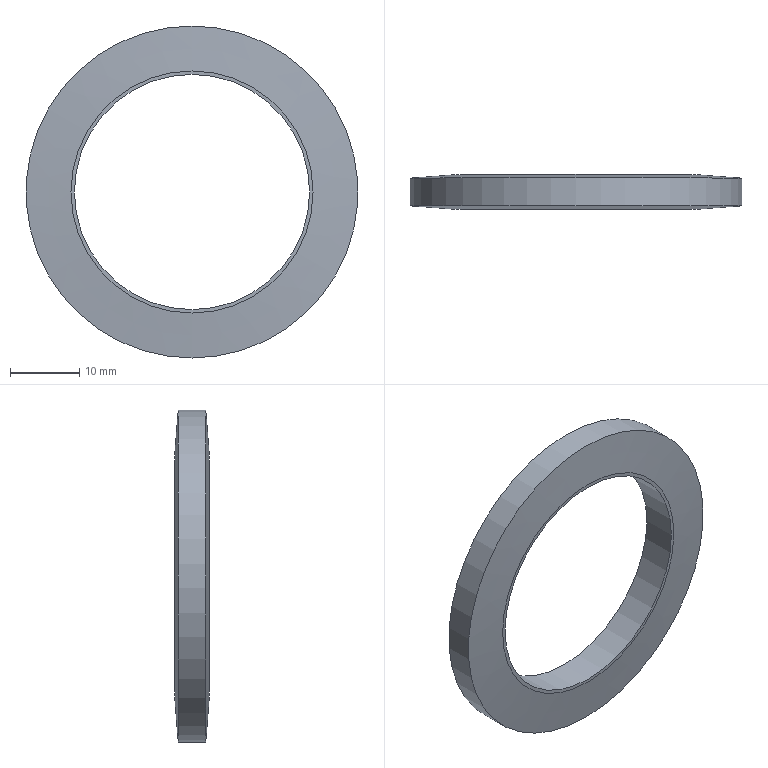Component | NX | FELT_RING_2 | 1 solid | 6 faces | box 48 x 5 x 48 mm | volume 4062 mm3 | cylinder 2 | plane 2 | cone 2 | commonest cylinder face diameters 48 x1 34 x1
STEP:
#1=CARTESIAN_POINT('',(0.,0.,0.));
#2=DIRECTION('',(0.,0.,1.));
#3=DIRECTION('',(1.,0.,0.));
#4=AXIS2_PLACEMENT_3D('',#1,#2,#3);
#5=CARTESIAN_POINT('',(378.803,-112.,-159.));
#6=VERTEX_POINT('',#5);
#7=CARTESIAN_POINT('',(378.803,-112.,-135.));
#8=DIRECTION('',(0.,-1.,0.));
#9=DIRECTION('',(0.,0.,-1.));
#10=AXIS2_PLACEMENT_3D('',#7,#8,#9);
#11=CIRCLE('',#10,24.);
#12=CARTESIAN_POINT('',(378.803,-116.5,-135.));
#13=DIRECTION('',(0.,1.,0.));
#14=DIRECTION('',(0.,0.,1.));
#15=AXIS2_PLACEMENT_3D('',#12,#13,#14);
#16=CYLINDRICAL_SURFACE('',#15,24.);
#17=CARTESIAN_POINT('',(9.425,4.5));
#18=DIRECTION('',(-1.,0.));
#19=VECTOR('',#18,1.);
#20=LINE('',#17,#19);
#21=(GEOMETRIC_REPRESENTATION_CONTEXT(2)PARAMETRIC_REPRESENTATION_CONTEXT()REPRESENTATION_CONTEXT('',''));
#22=DEFINITIONAL_REPRESENTATION('',(#20),#21);
#23=PCURVE('',#16,#22);
#24=CARTESIAN_POINT('',(378.803,-112.,-135.));
#25=DIRECTION('',(0.,-1.,0.));
#26=DIRECTION('',(0.,0.,-1.));
#27=AXIS2_PLACEMENT_3D('',#24,#25,#26);
#28=CONICAL_SURFACE('',#27,24.,1.494);
#29=CARTESIAN_POINT('',(0.,0.));
#30=DIRECTION('',(1.,0.));
#31=VECTOR('',#30,1.);
#32=LINE('',#29,#31);
#33=(GEOMETRIC_REPRESENTATION_CONTEXT(2)PARAMETRIC_REPRESENTATION_CONTEXT()REPRESENTATION_CONTEXT('',''));
#34=DEFINITIONAL_REPRESENTATION('',(#32),#33);
#35=PCURVE('',#28,#34);
#36=SURFACE_CURVE('',#11,(#23,#35),.PCURVE_S1.);
#37=EDGE_CURVE('',#6,#6,#36,.T.);
#38=ORIENTED_EDGE('',*,*,#37,.T.);
#39=CARTESIAN_POINT('',(378.803,-116.,-159.));
#40=VERTEX_POINT('',#39);
#41=CARTESIAN_POINT('',(378.803,-116.,-159.));
#42=CARTESIAN_POINT('',(378.803,-112.,-159.));
#43=B_SPLINE_CURVE_WITH_KNOTS('',1,(#41,#42),.UNSPECIFIED.,.F.,.F.,(2,2),(0.5,4.5),.PIECEWISE_BEZIER_KNOTS.);
#44=CARTESIAN_POINT('',(3.142,0.));
#45=DIRECTION('',(0.,1.));
#46=VECTOR('',#45,1.);
#47=LINE('',#44,#46);
#48=(GEOMETRIC_REPRESENTATION_CONTEXT(2)PARAMETRIC_REPRESENTATION_CONTEXT()REPRESENTATION_CONTEXT('',''));
#49=DEFINITIONAL_REPRESENTATION('',(#47),#48);
#50=PCURVE('',#16,#49);
#51=CARTESIAN_POINT('',(9.425,0.));
#52=DIRECTION('',(0.,1.));
#53=VECTOR('',#52,1.);
#54=LINE('',#51,#53);
#55=(GEOMETRIC_REPRESENTATION_CONTEXT(2)PARAMETRIC_REPRESENTATION_CONTEXT()REPRESENTATION_CONTEXT('',''));
#56=DEFINITIONAL_REPRESENTATION('',(#54),#55);
#57=PCURVE('',#16,#56);
#58=SEAM_CURVE('',#43,(#50,#57),.PCURVE_S1.);
#59=EDGE_CURVE('',#40,#6,#58,.T.);
#60=ORIENTED_EDGE('',*,*,#59,.F.);
#61=CARTESIAN_POINT('',(378.803,-116.,-135.));
#62=DIRECTION('',(0.,1.,0.));
#63=DIRECTION('',(0.,0.,-1.));
#64=AXIS2_PLACEMENT_3D('',#61,#62,#63);
#65=CIRCLE('',#64,24.);
#66=CARTESIAN_POINT('',(3.142,0.5));
#67=DIRECTION('',(1.,0.));
#68=VECTOR('',#67,1.);
#69=LINE('',#66,#68);
#70=(GEOMETRIC_REPRESENTATION_CONTEXT(2)PARAMETRIC_REPRESENTATION_CONTEXT()REPRESENTATION_CONTEXT('',''));
#71=DEFINITIONAL_REPRESENTATION('',(#69),#70);
#72=PCURVE('',#16,#71);
#73=CARTESIAN_POINT('',(378.803,-116.5,-135.));
#74=DIRECTION('',(0.,1.,0.));
#75=DIRECTION('',(0.,0.,1.));
#76=AXIS2_PLACEMENT_3D('',#73,#74,#75);
#77=CONICAL_SURFACE('',#76,17.5,1.494);
#78=CARTESIAN_POINT('',(3.142,0.5));
#79=DIRECTION('',(1.,0.));
#80=VECTOR('',#79,1.);
#81=LINE('',#78,#80);
#82=(GEOMETRIC_REPRESENTATION_CONTEXT(2)PARAMETRIC_REPRESENTATION_CONTEXT()REPRESENTATION_CONTEXT('',''));
#83=DEFINITIONAL_REPRESENTATION('',(#81),#82);
#84=PCURVE('',#77,#83);
#85=SURFACE_CURVE('',#65,(#72,#84),.PCURVE_S1.);
#86=EDGE_CURVE('',#40,#40,#85,.T.);
#87=ORIENTED_EDGE('',*,*,#86,.T.);
#88=ORIENTED_EDGE('',*,*,#59,.T.);
#89=EDGE_LOOP('',(#38,#60,#87,#88));
#90=FACE_BOUND('',#89,.T.);
#91=ADVANCED_FACE('',(#90),#16,.T.);
#92=CARTESIAN_POINT('',(395.803,-116.5,-135.));
#93=VERTEX_POINT('',#92);
#94=CARTESIAN_POINT('',(378.803,-116.5,-135.));
#95=DIRECTION('',(0.,-1.,0.));
#96=DIRECTION('',(1.,0.,0.));
#97=AXIS2_PLACEMENT_3D('',#94,#95,#96);
#98=CIRCLE('',#97,17.);
#99=CARTESIAN_POINT('',(378.803,-116.5,-135.));
#100=DIRECTION('',(0.,1.,0.));
#101=DIRECTION('',(0.,0.,1.));
#102=AXIS2_PLACEMENT_3D('',#99,#100,#101);
#103=CYLINDRICAL_SURFACE('',#102,17.);
#104=CARTESIAN_POINT('',(7.854,0.));
#105=DIRECTION('',(-1.,0.));
#106=VECTOR('',#105,1.);
#107=LINE('',#104,#106);
#108=(GEOMETRIC_REPRESENTATION_CONTEXT(2)PARAMETRIC_REPRESENTATION_CONTEXT()REPRESENTATION_CONTEXT('',''));
#109=DEFINITIONAL_REPRESENTATION('',(#107),#108);
#110=PCURVE('',#103,#109);
#111=CARTESIAN_POINT('',(378.803,-116.5,-135.));
#112=DIRECTION('',(0.,-1.,0.));
#113=DIRECTION('',(0.,0.,-1.));
#114=AXIS2_PLACEMENT_3D('',#111,#112,#113);
#115=PLANE('',#114);
#116=CARTESIAN_POINT('',(0.,0.));
#117=DIRECTION('',(0.,1.));
#118=AXIS2_PLACEMENT_2D('',#116,#117);
#119=CIRCLE('',#118,17.);
#120=(GEOMETRIC_REPRESENTATION_CONTEXT(2)PARAMETRIC_REPRESENTATION_CONTEXT()REPRESENTATION_CONTEXT('',''));
#121=DEFINITIONAL_REPRESENTATION('',(#119),#120);
#122=PCURVE('',#115,#121);
#123=SURFACE_CURVE('',#98,(#110,#122),.PCURVE_S1.);
#124=EDGE_CURVE('',#93,#93,#123,.T.);
#125=ORIENTED_EDGE('',*,*,#124,.F.);
#126=CARTESIAN_POINT('',(395.803,-111.5,-135.));
#127=VERTEX_POINT('',#126);
#128=CARTESIAN_POINT('',(395.803,-116.5,-135.));
#129=CARTESIAN_POINT('',(395.803,-111.5,-135.));
#130=B_SPLINE_CURVE_WITH_KNOTS('',1,(#128,#129),.UNSPECIFIED.,.F.,.F.,(2,2),(0.,5.),.PIECEWISE_BEZIER_KNOTS.);
#131=CARTESIAN_POINT('',(7.854,0.));
#132=DIRECTION('',(0.,1.));
#133=VECTOR('',#132,1.);
#134=LINE('',#131,#133);
#135=(GEOMETRIC_REPRESENTATION_CONTEXT(2)PARAMETRIC_REPRESENTATION_CONTEXT()REPRESENTATION_CONTEXT('',''));
#136=DEFINITIONAL_REPRESENTATION('',(#134),#135);
#137=PCURVE('',#103,#136);
#138=CARTESIAN_POINT('',(1.571,0.));
#139=DIRECTION('',(0.,1.));
#140=VECTOR('',#139,1.);
#141=LINE('',#138,#140);
#142=(GEOMETRIC_REPRESENTATION_CONTEXT(2)PARAMETRIC_REPRESENTATION_CONTEXT()REPRESENTATION_CONTEXT('',''));
#143=DEFINITIONAL_REPRESENTATION('',(#141),#142);
#144=PCURVE('',#103,#143);
#145=SEAM_CURVE('',#130,(#137,#144),.PCURVE_S1.);
#146=EDGE_CURVE('',#93,#127,#145,.T.);
#147=ORIENTED_EDGE('',*,*,#146,.T.);
#148=CARTESIAN_POINT('',(378.803,-111.5,-135.));
#149=DIRECTION('',(0.,-1.,0.));
#150=DIRECTION('',(1.,0.,0.));
#151=AXIS2_PLACEMENT_3D('',#148,#149,#150);
#152=CIRCLE('',#151,17.);
#153=CARTESIAN_POINT('',(7.854,5.));
#154=DIRECTION('',(-1.,0.));
#155=VECTOR('',#154,1.);
#156=LINE('',#153,#155);
#157=(GEOMETRIC_REPRESENTATION_CONTEXT(2)PARAMETRIC_REPRESENTATION_CONTEXT()REPRESENTATION_CONTEXT('',''));
#158=DEFINITIONAL_REPRESENTATION('',(#156),#157);
#159=PCURVE('',#103,#158);
#160=CARTESIAN_POINT('',(378.803,-111.5,-135.));
#161=DIRECTION('',(0.,-1.,0.));
#162=DIRECTION('',(0.,0.,-1.));
#163=AXIS2_PLACEMENT_3D('',#160,#161,#162);
#164=PLANE('',#163);
#165=CARTESIAN_POINT('',(0.,0.));
#166=DIRECTION('',(0.,1.));
#167=AXIS2_PLACEMENT_2D('',#165,#166);
#168=CIRCLE('',#167,17.);
#169=(GEOMETRIC_REPRESENTATION_CONTEXT(2)PARAMETRIC_REPRESENTATION_CONTEXT()REPRESENTATION_CONTEXT('',''));
#170=DEFINITIONAL_REPRESENTATION('',(#168),#169);
#171=PCURVE('',#164,#170);
#172=SURFACE_CURVE('',#152,(#159,#171),.PCURVE_S1.);
#173=EDGE_CURVE('',#127,#127,#172,.T.);
#174=ORIENTED_EDGE('',*,*,#173,.T.);
#175=ORIENTED_EDGE('',*,*,#146,.F.);
#176=EDGE_LOOP('',(#125,#147,#174,#175));
#177=FACE_BOUND('',#176,.F.);
#178=ADVANCED_FACE('',(#177),#103,.F.);
#179=CARTESIAN_POINT('',(378.803,-116.5,-152.5));
#180=VERTEX_POINT('',#179);
#181=CARTESIAN_POINT('',(378.803,-116.5,-135.));
#182=DIRECTION('',(0.,-1.,0.));
#183=DIRECTION('',(0.,0.,-1.));
#184=AXIS2_PLACEMENT_3D('',#181,#182,#183);
#185=CIRCLE('',#184,17.5);
#186=CARTESIAN_POINT('',(0.,0.));
#187=DIRECTION('',(1.,0.));
#188=AXIS2_PLACEMENT_2D('',#186,#187);
#189=CIRCLE('',#188,17.5);
#190=(GEOMETRIC_REPRESENTATION_CONTEXT(2)PARAMETRIC_REPRESENTATION_CONTEXT()REPRESENTATION_CONTEXT('',''));
#191=DEFINITIONAL_REPRESENTATION('',(#189),#190);
#192=PCURVE('',#115,#191);
#193=CARTESIAN_POINT('',(9.425,0.));
#194=DIRECTION('',(-1.,0.));
#195=VECTOR('',#194,1.);
#196=LINE('',#193,#195);
#197=(GEOMETRIC_REPRESENTATION_CONTEXT(2)PARAMETRIC_REPRESENTATION_CONTEXT()REPRESENTATION_CONTEXT('',''));
#198=DEFINITIONAL_REPRESENTATION('',(#196),#197);
#199=PCURVE('',#77,#198);
#200=SURFACE_CURVE('',#185,(#192,#199),.PCURVE_S1.);
#201=EDGE_CURVE('',#180,#180,#200,.T.);
#202=ORIENTED_EDGE('',*,*,#201,.T.);
#203=EDGE_LOOP('',(#202));
#204=FACE_BOUND('',#203,.T.);
#205=ORIENTED_EDGE('',*,*,#124,.F.);
#206=EDGE_LOOP('',(#205));
#207=FACE_BOUND('',#206,.T.);
#208=ADVANCED_FACE('',(#204,#207),#115,.T.);
#209=CARTESIAN_POINT('',(378.803,-111.5,-152.5));
#210=VERTEX_POINT('',#209);
#211=CARTESIAN_POINT('',(378.803,-111.5,-135.));
#212=DIRECTION('',(0.,1.,0.));
#213=DIRECTION('',(0.,0.,-1.));
#214=AXIS2_PLACEMENT_3D('',#211,#212,#213);
#215=CIRCLE('',#214,17.5);
#216=CARTESIAN_POINT('',(17.5,0.));
#217=CARTESIAN_POINT('',(17.5,-30.311));
#218=CARTESIAN_POINT('',(-8.75,-15.155));
#219=CARTESIAN_POINT('',(-35.,-0.));
#220=CARTESIAN_POINT('',(-8.75,15.155));
#221=CARTESIAN_POINT('',(17.5,30.311));
#222=CARTESIAN_POINT('',(17.5,0.));
#223=(BOUNDED_CURVE()B_SPLINE_CURVE(2,(#216,#217,#218,#219,#220,#221,#222),.UNSPECIFIED.,.T.,.F.)B_SPLINE_CURVE_WITH_KNOTS((1,2,2,2,2,1),(-2.094,0.,2.094,4.189,6.283,8.378),.UNSPECIFIED.)CURVE()GEOMETRIC_REPRESENTATION_ITEM()RATIONAL_B_SPLINE_CURVE((1.,0.5,1.,0.5,1.,0.5,1.))REPRESENTATION_ITEM(''));
#224=(GEOMETRIC_REPRESENTATION_CONTEXT(2)PARAMETRIC_REPRESENTATION_CONTEXT()REPRESENTATION_CONTEXT('',''));
#225=DEFINITIONAL_REPRESENTATION('',(#223),#224);
#226=PCURVE('',#164,#225);
#227=CARTESIAN_POINT('',(6.283,-0.5));
#228=DIRECTION('',(-1.,0.));
#229=VECTOR('',#228,1.);
#230=LINE('',#227,#229);
#231=(GEOMETRIC_REPRESENTATION_CONTEXT(2)PARAMETRIC_REPRESENTATION_CONTEXT()REPRESENTATION_CONTEXT('',''));
#232=DEFINITIONAL_REPRESENTATION('',(#230),#231);
#233=PCURVE('',#28,#232);
#234=SURFACE_CURVE('',#215,(#226,#233),.PCURVE_S1.);
#235=EDGE_CURVE('',#210,#210,#234,.T.);
#236=ORIENTED_EDGE('',*,*,#235,.T.);
#237=EDGE_LOOP('',(#236));
#238=FACE_BOUND('',#237,.T.);
#239=ORIENTED_EDGE('',*,*,#173,.T.);
#240=EDGE_LOOP('',(#239));
#241=FACE_BOUND('',#240,.T.);
#242=ADVANCED_FACE('',(#238,#241),#164,.F.);
#243=ORIENTED_EDGE('',*,*,#86,.F.);
#244=CARTESIAN_POINT('',(378.803,-116.5,-152.5));
#245=CARTESIAN_POINT('',(378.803,-116.,-159.));
#246=B_SPLINE_CURVE_WITH_KNOTS('',1,(#244,#245),.UNSPECIFIED.,.F.,.F.,(2,2),(0.,6.519),.PIECEWISE_BEZIER_KNOTS.);
#247=CARTESIAN_POINT('',(3.142,0.));
#248=DIRECTION('',(0.,1.));
#249=VECTOR('',#248,1.);
#250=LINE('',#247,#249);
#251=(GEOMETRIC_REPRESENTATION_CONTEXT(2)PARAMETRIC_REPRESENTATION_CONTEXT()REPRESENTATION_CONTEXT('',''));
#252=DEFINITIONAL_REPRESENTATION('',(#250),#251);
#253=PCURVE('',#77,#252);
#254=CARTESIAN_POINT('',(9.425,0.));
#255=DIRECTION('',(0.,1.));
#256=VECTOR('',#255,1.);
#257=LINE('',#254,#256);
#258=(GEOMETRIC_REPRESENTATION_CONTEXT(2)PARAMETRIC_REPRESENTATION_CONTEXT()REPRESENTATION_CONTEXT('',''));
#259=DEFINITIONAL_REPRESENTATION('',(#257),#258);
#260=PCURVE('',#77,#259);
#261=SEAM_CURVE('',#246,(#253,#260),.PCURVE_S1.);
#262=EDGE_CURVE('',#180,#40,#261,.T.);
#263=ORIENTED_EDGE('',*,*,#262,.F.);
#264=ORIENTED_EDGE('',*,*,#201,.F.);
#265=ORIENTED_EDGE('',*,*,#262,.T.);
#266=EDGE_LOOP('',(#243,#263,#264,#265));
#267=FACE_BOUND('',#266,.T.);
#268=ADVANCED_FACE('',(#267),#77,.T.);
#269=ORIENTED_EDGE('',*,*,#235,.F.);
#270=CARTESIAN_POINT('',(378.803,-111.5,-152.5));
#271=CARTESIAN_POINT('',(378.803,-112.,-159.));
#272=B_SPLINE_CURVE_WITH_KNOTS('',1,(#270,#271),.UNSPECIFIED.,.F.,.F.,(2,2),(-6.519,0.),.PIECEWISE_BEZIER_KNOTS.);
#273=CARTESIAN_POINT('',(6.283,0.));
#274=DIRECTION('',(0.,1.));
#275=VECTOR('',#274,1.);
#276=LINE('',#273,#275);
#277=(GEOMETRIC_REPRESENTATION_CONTEXT(2)PARAMETRIC_REPRESENTATION_CONTEXT()REPRESENTATION_CONTEXT('',''));
#278=DEFINITIONAL_REPRESENTATION('',(#276),#277);
#279=PCURVE('',#28,#278);
#280=CARTESIAN_POINT('',(0.,0.));
#281=DIRECTION('',(0.,1.));
#282=VECTOR('',#281,1.);
#283=LINE('',#280,#282);
#284=(GEOMETRIC_REPRESENTATION_CONTEXT(2)PARAMETRIC_REPRESENTATION_CONTEXT()REPRESENTATION_CONTEXT('',''));
#285=DEFINITIONAL_REPRESENTATION('',(#283),#284);
#286=PCURVE('',#28,#285);
#287=SEAM_CURVE('',#272,(#279,#286),.PCURVE_S1.);
#288=EDGE_CURVE('',#210,#6,#287,.T.);
#289=ORIENTED_EDGE('',*,*,#288,.T.);
#290=ORIENTED_EDGE('',*,*,#37,.F.);
#291=ORIENTED_EDGE('',*,*,#288,.F.);
#292=EDGE_LOOP('',(#269,#289,#290,#291));
#293=FACE_BOUND('',#292,.T.);
#294=ADVANCED_FACE('',(#293),#28,.T.);
#295=CLOSED_SHELL('',(#91,#178,#208,#242,#268,#294));
#296=MANIFOLD_SOLID_BREP('',#295);
#297=(LENGTH_UNIT()NAMED_UNIT(*)SI_UNIT(.MILLI.,.METRE.));
#298=UNCERTAINTY_MEASURE_WITH_UNIT(LENGTH_MEASURE(0.00001),#297,'','');
#299=(NAMED_UNIT(*)PLANE_ANGLE_UNIT()SI_UNIT($,.RADIAN.));
#300=(NAMED_UNIT(*)SI_UNIT($,.STERADIAN.)SOLID_ANGLE_UNIT());
#301=(GEOMETRIC_REPRESENTATION_CONTEXT(3)GLOBAL_UNCERTAINTY_ASSIGNED_CONTEXT((#298))GLOBAL_UNIT_ASSIGNED_CONTEXT((#297,#299,#300))REPRESENTATION_CONTEXT('',''));
#302=ADVANCED_BREP_SHAPE_REPRESENTATION('',(#4,#296),#301);